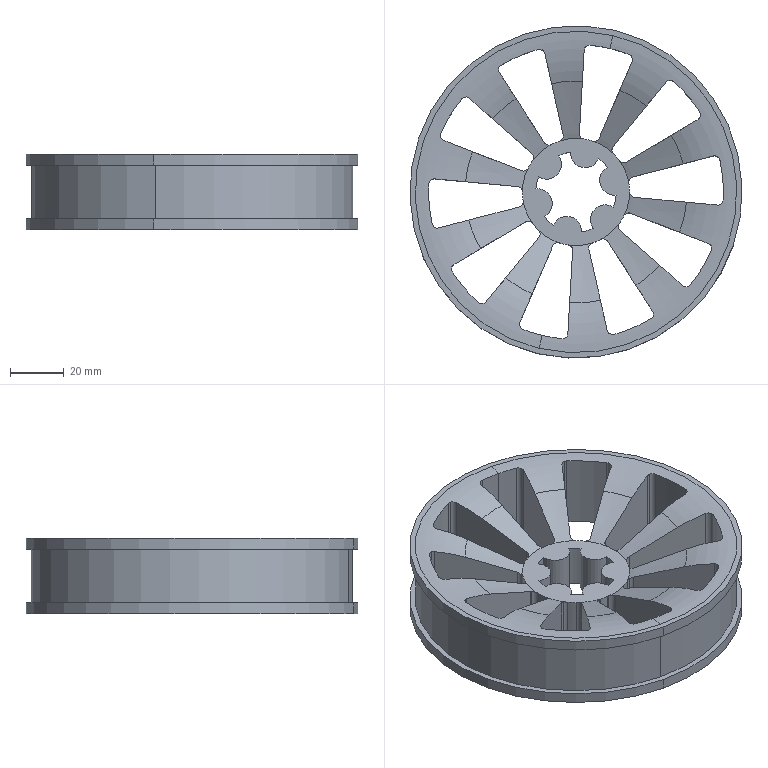Component | SolidWorks | DriveDevice-1_DriveWheel-1 | 1 solid | 130 faces | volume 156868 mm3 | cylinder 93 | plane 25 | cone 10 | torus 2 | commonest cylinder face diameters 4 x50 110 x11 40 x11 11 x9 30 x6 124 x4 120 x2